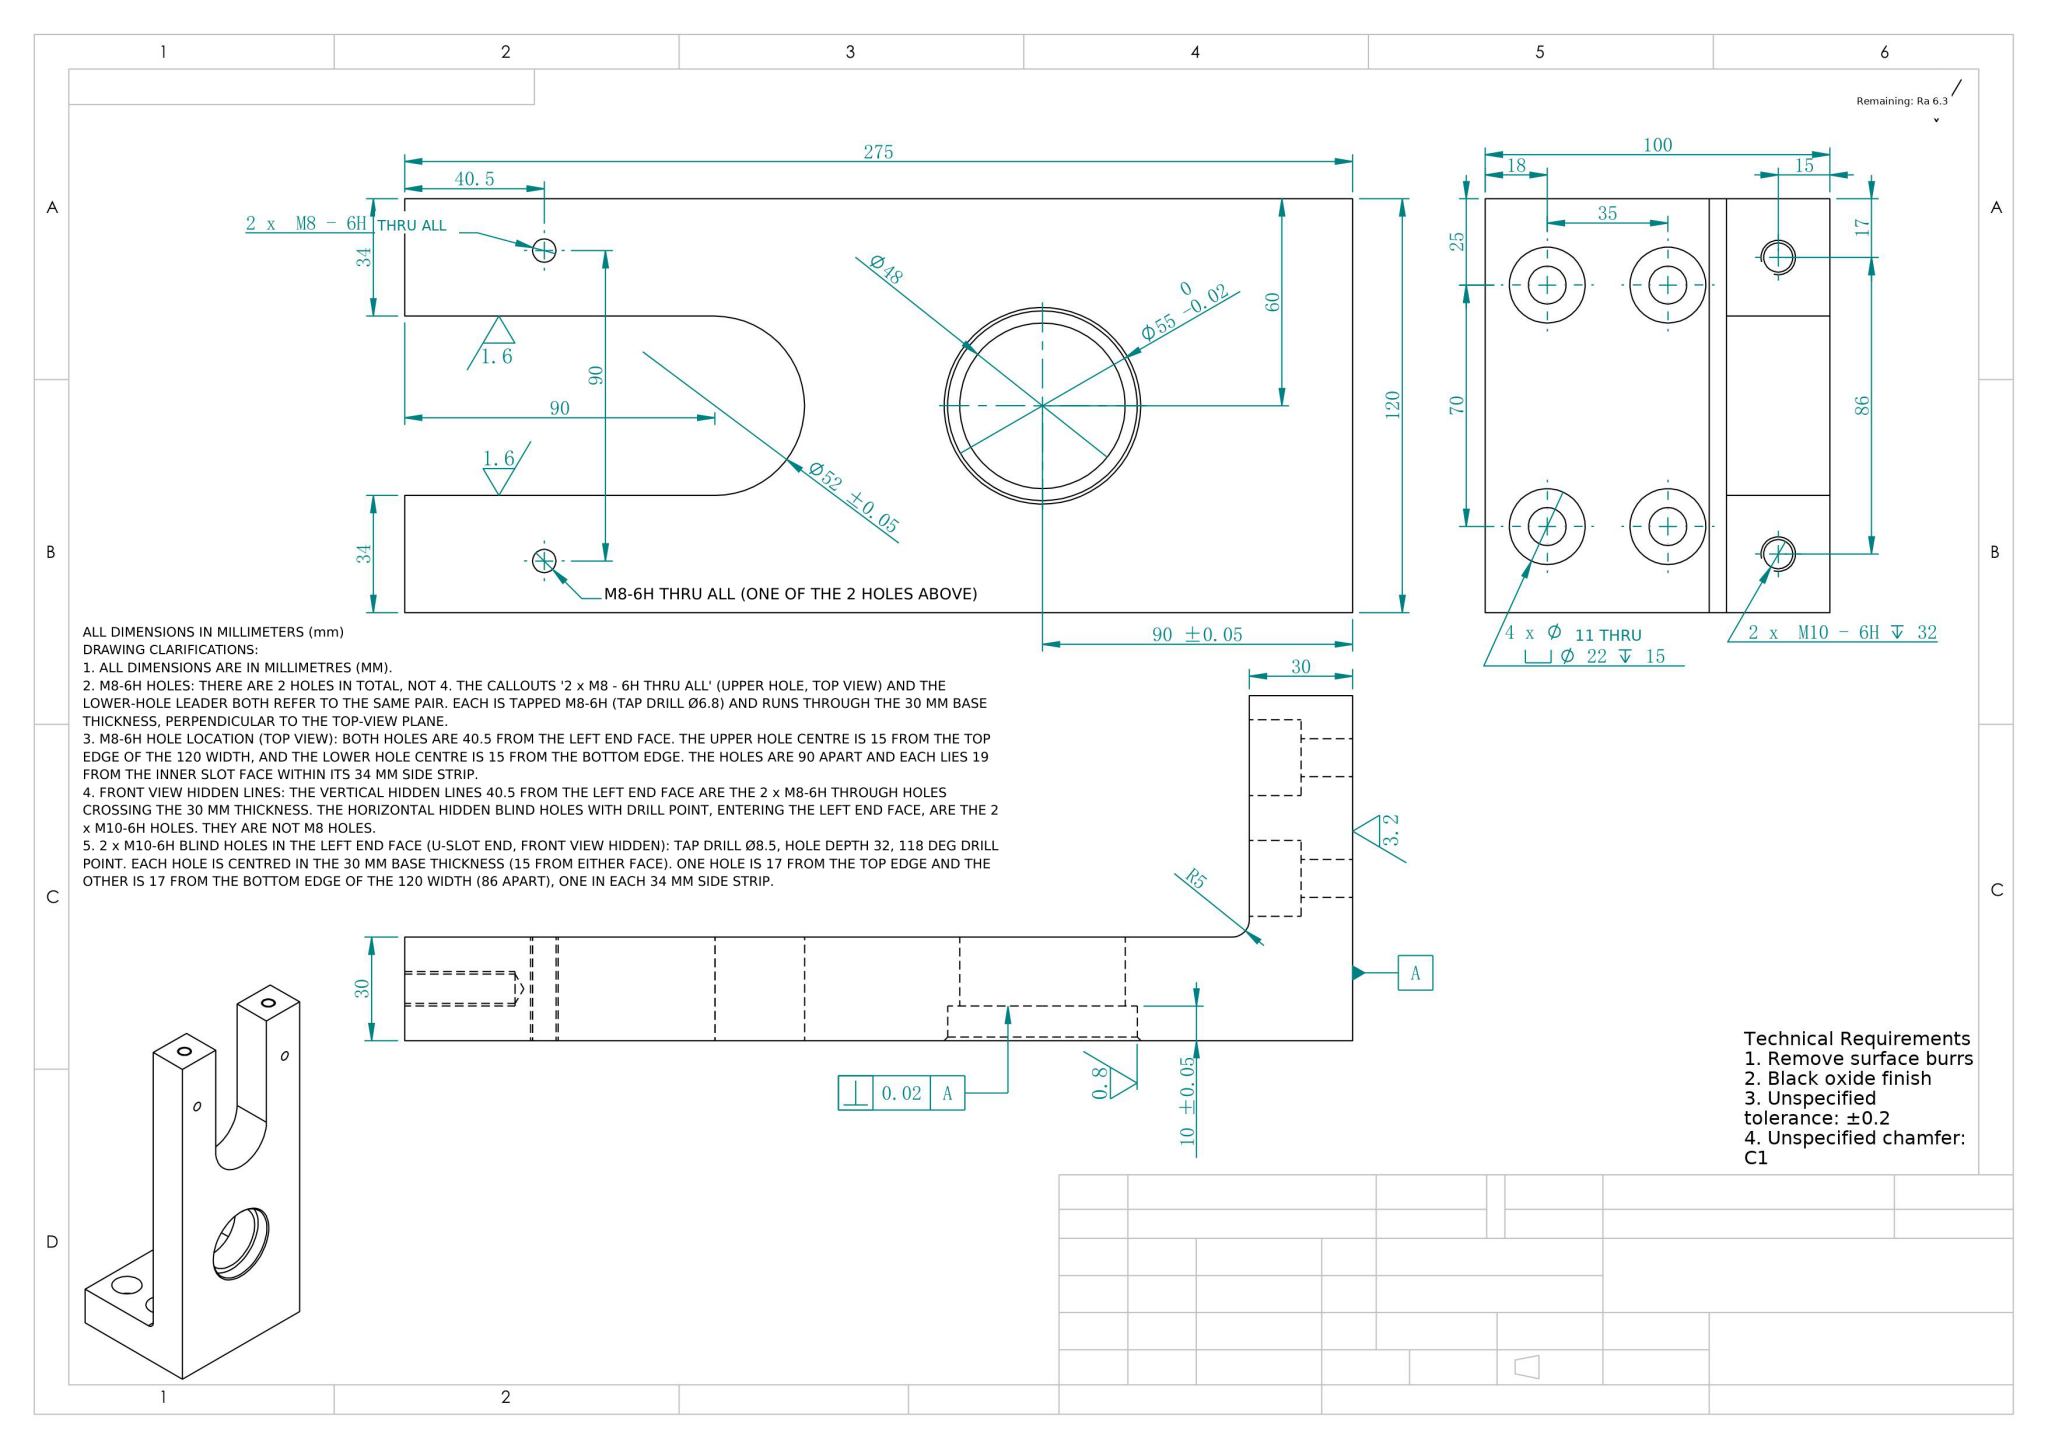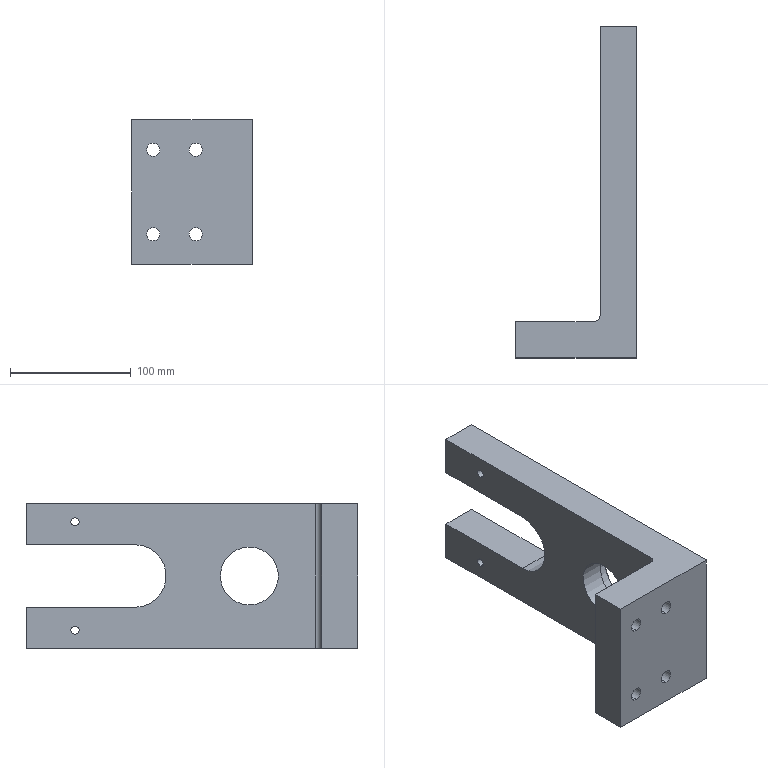Part | NX | mm | Slotted Right-Angle Bearing Mount | 1 solid | 52 faces | box 100 x 275 x 120 mm | volume 975934 mm3 | cylinder 30 | plane 16 | cone 6 | commonest cylinder face diameters 22 x8 11 x8 8.5 x4 6.8 x4 48 x2 55 x2 52 x1 10 x1